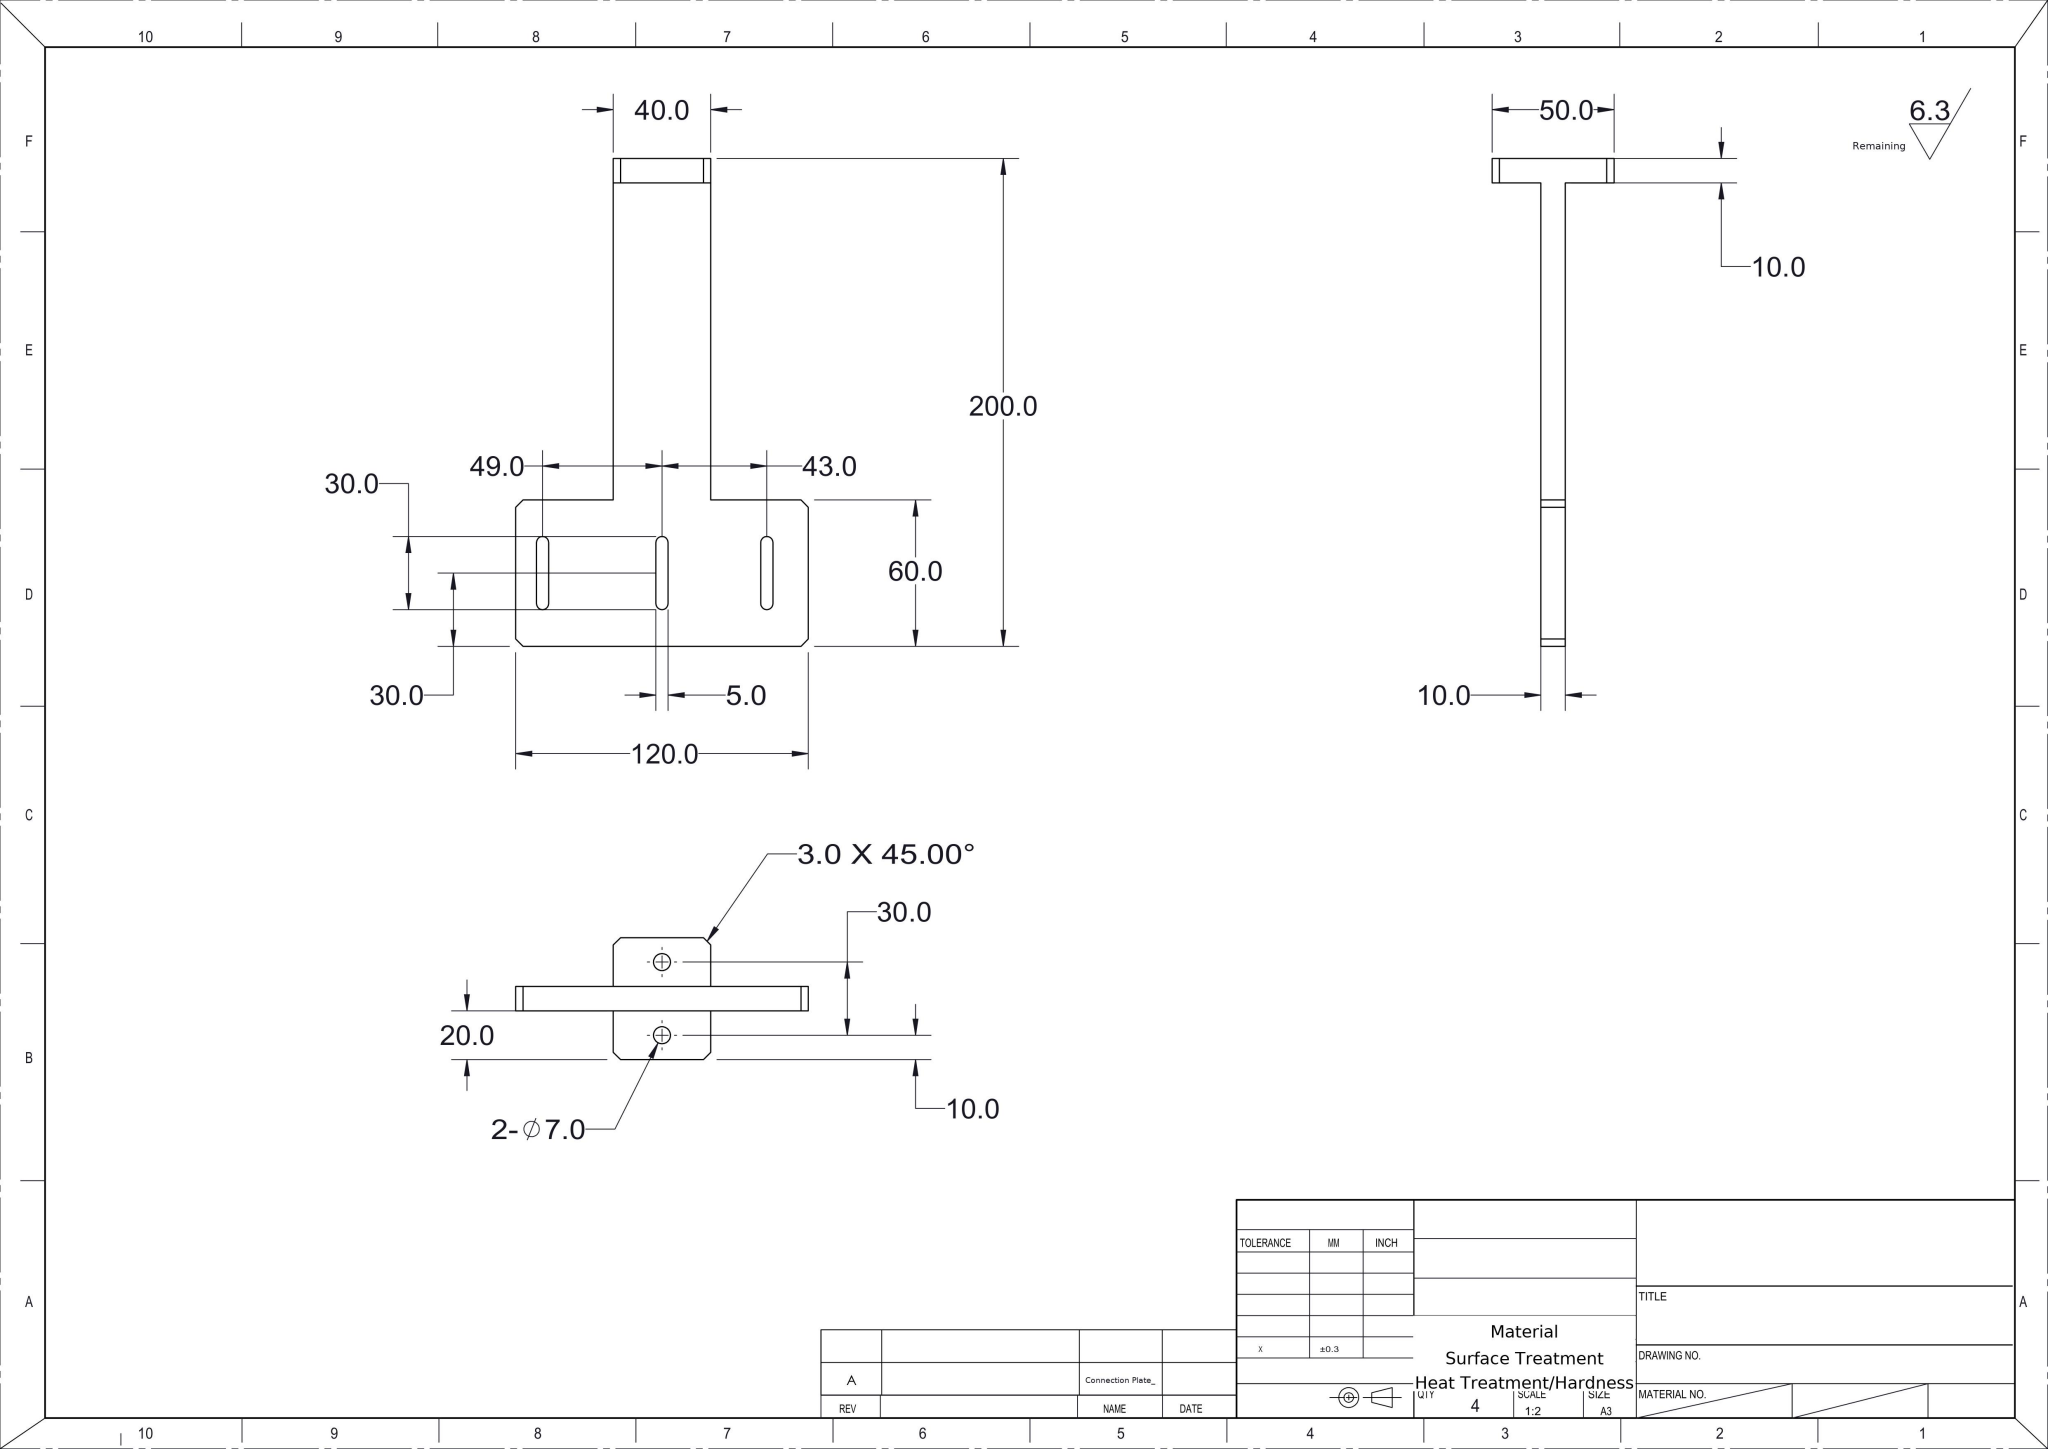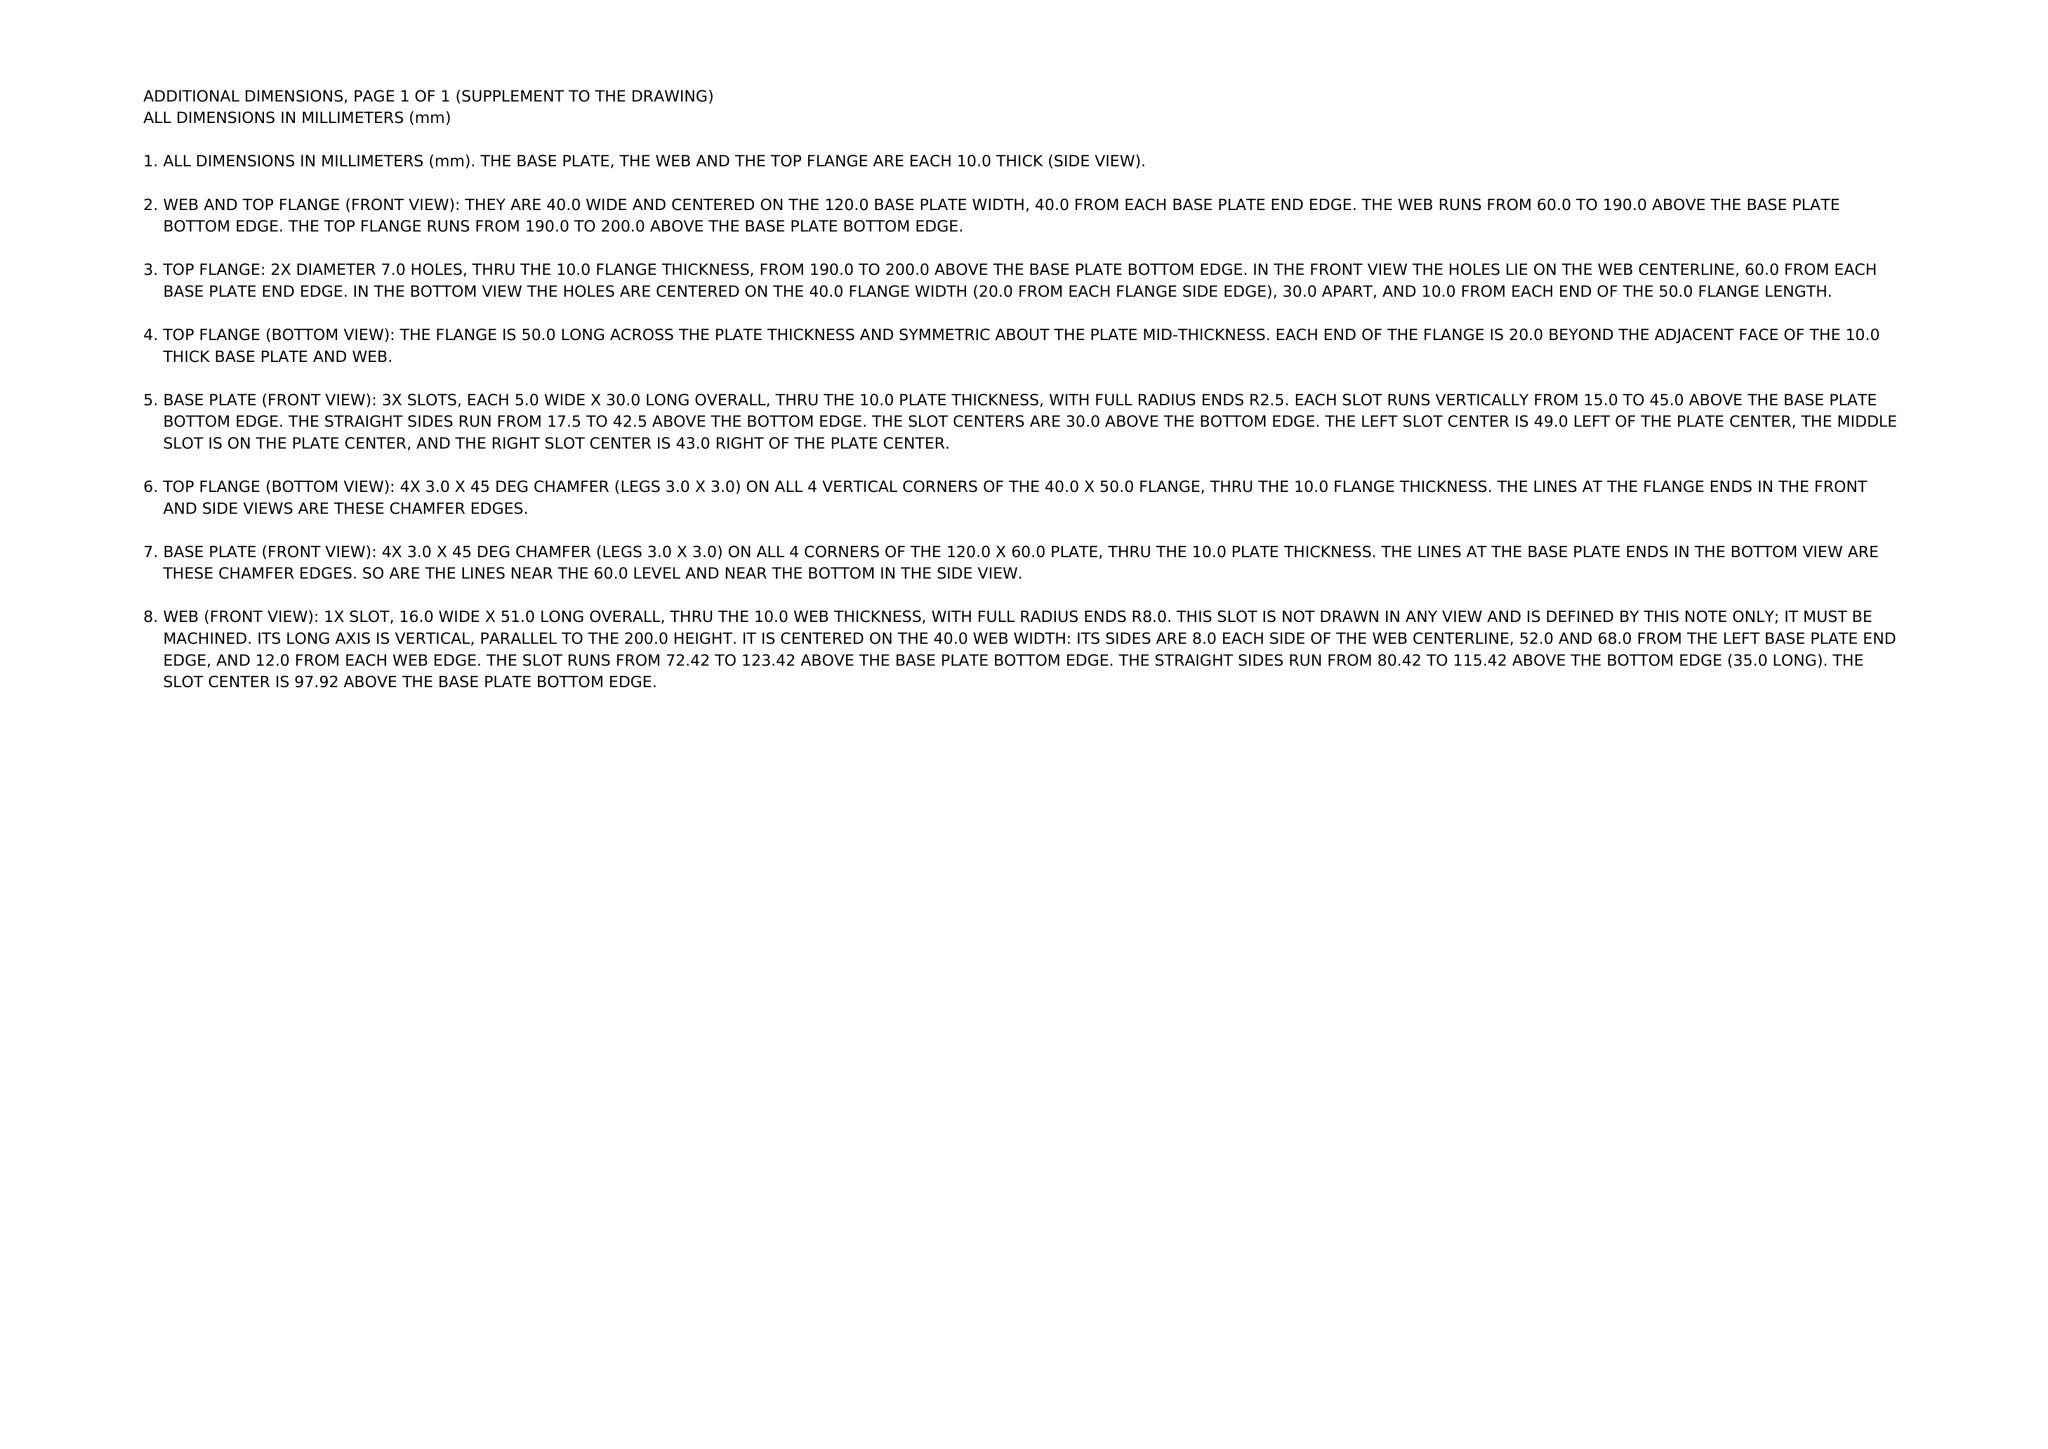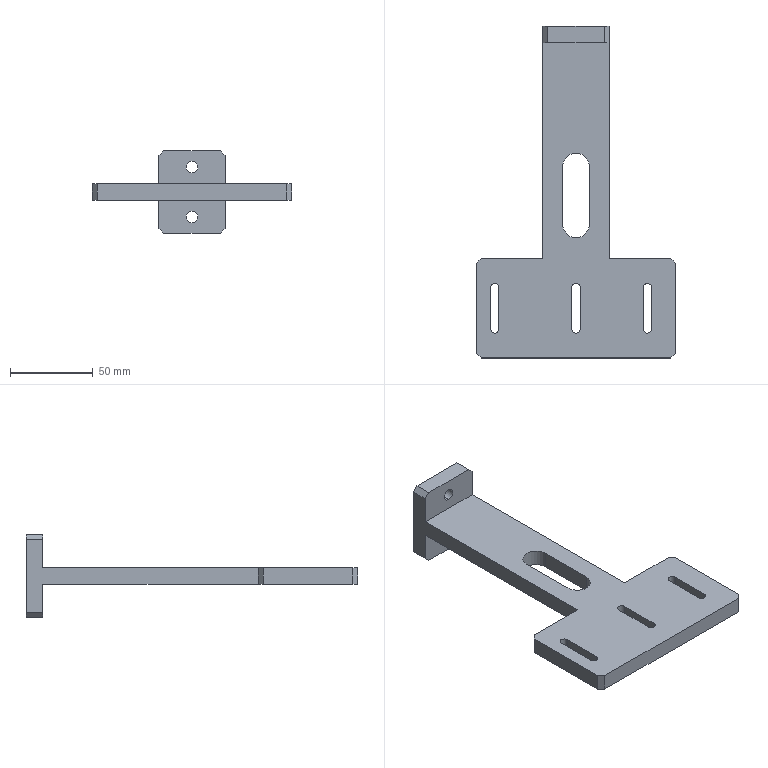Part | NX | mm | 1 solid | 42 faces | box 120 x 200 x 50 mm | volume 130921 mm3 | plane 30 | cylinder 12 | commonest cylinder face diameters 5 x6 7 x4 16 x2